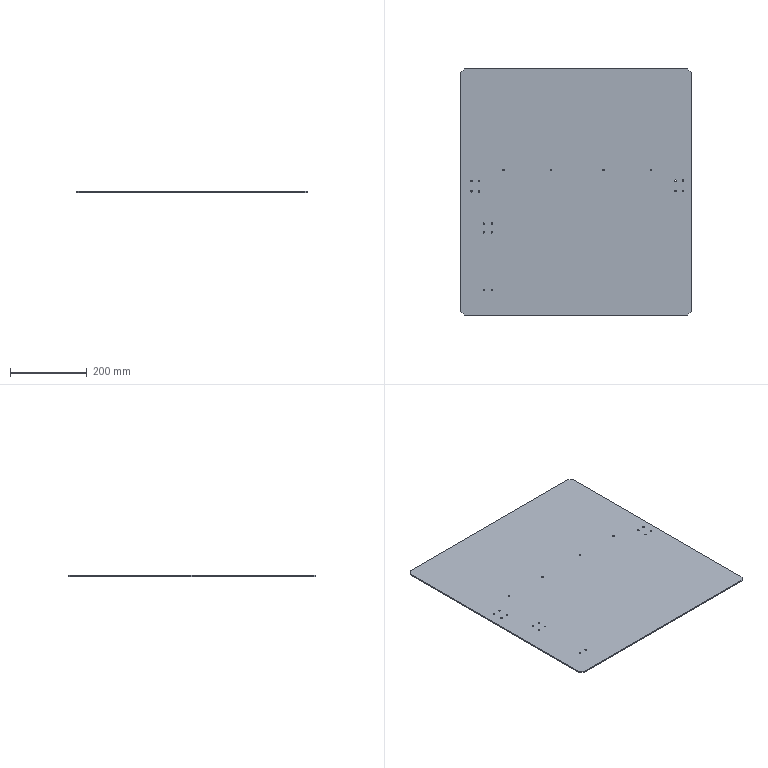Component | SolidWorks | 01-01FrameBody-1_04CounterweightPlate-4 | 1 solid | 46 faces | box 600 x 640 x 3 mm | volume 1150747 mm3 | cylinder 36 | plane 10 | commonest cylinder face diameters 4.2 x24 3.3 x12 | material 4040 Square Tube
build123d program:
from build123d import *

# Parameters (mm, degrees)
SKETCH1_W             = 600
SKETCH1_H             = 640
BOSS_EXTRUDE1_DEPTH   = 3
CHAMFER1_SIZE         = 10
M5_TAPPED_HOLE1_D     = 4.2
M5_TAPPED_HOLE1_DEPTH = 14
M5_TAPPED_HOLE1_TIP   = 1.262
M4_TAPPED_HOLE1_D     = 3.3
M4_TAPPED_HOLE1_DEPTH = 11.5
M4_TAPPED_HOLE1_TIP   = 0.9914


with BuildPart() as part:
    # Sketch1 → Boss-Extrude1 (new body)
    with BuildSketch(Plane(origin=(0, 0, 0), x_dir=(1, 0, 0), z_dir=(0, 1, 0))):
        Rectangle(SKETCH1_W, SKETCH1_H)
    extrude(amount=BOSS_EXTRUDE1_DEPTH)

    # Chamfer1
    chamfer1_edges = [part.edges().sort_by_distance(p)[0] for p in [
        (-300, 1.5, -320),
        (300, 1.5, -320),
        (300, 1.5, 320),
        (-300, 1.5, 320),
    ]]
    chamfer(chamfer1_edges, length=CHAMFER1_SIZE)

    # M5 Tapped Hole1
    with Locations(Plane(origin=(0, 3, 0), x_dir=(-1, 0, 0), z_dir=(0, 1, 0))):
        with Locations((-258.5, -29.5), (272, -29), (252, -29), (252, -2), (272, -2), (-194.75, -57), (-71.25, -57), (65.25, -57), (188.75, -57), (-258.5, -2.5), (-278.5, -2.5), (-278.5, -29.5)):
            Hole(M5_TAPPED_HOLE1_D / 2, depth=M5_TAPPED_HOLE1_DEPTH)
            with Locations((0, 0, -(M5_TAPPED_HOLE1_DEPTH + M5_TAPPED_HOLE1_TIP / 2))):  # 118° drill point
                Cone(0, M5_TAPPED_HOLE1_D / 2, M5_TAPPED_HOLE1_TIP, mode=Mode.SUBTRACT)

    # M4 Tapped Hole1
    with Locations(Plane(origin=(0, 3, 0), x_dir=(-1, 0, 0), z_dir=(0, 1, 0))):
        with Locations((240, 105), (219, 105), (219, 254), (240, 254), (240, 82), (219, 82)):
            Hole(M4_TAPPED_HOLE1_D / 2, depth=M4_TAPPED_HOLE1_DEPTH)
            with Locations((0, 0, -(M4_TAPPED_HOLE1_DEPTH + M4_TAPPED_HOLE1_TIP / 2))):  # 118° drill point
                Cone(0, M4_TAPPED_HOLE1_D / 2, M4_TAPPED_HOLE1_TIP, mode=Mode.SUBTRACT)


solid = part.part

# Placed as in the assembly
solid = solid.moved(Location((-340, 360, 52), (90, 0, 0)))